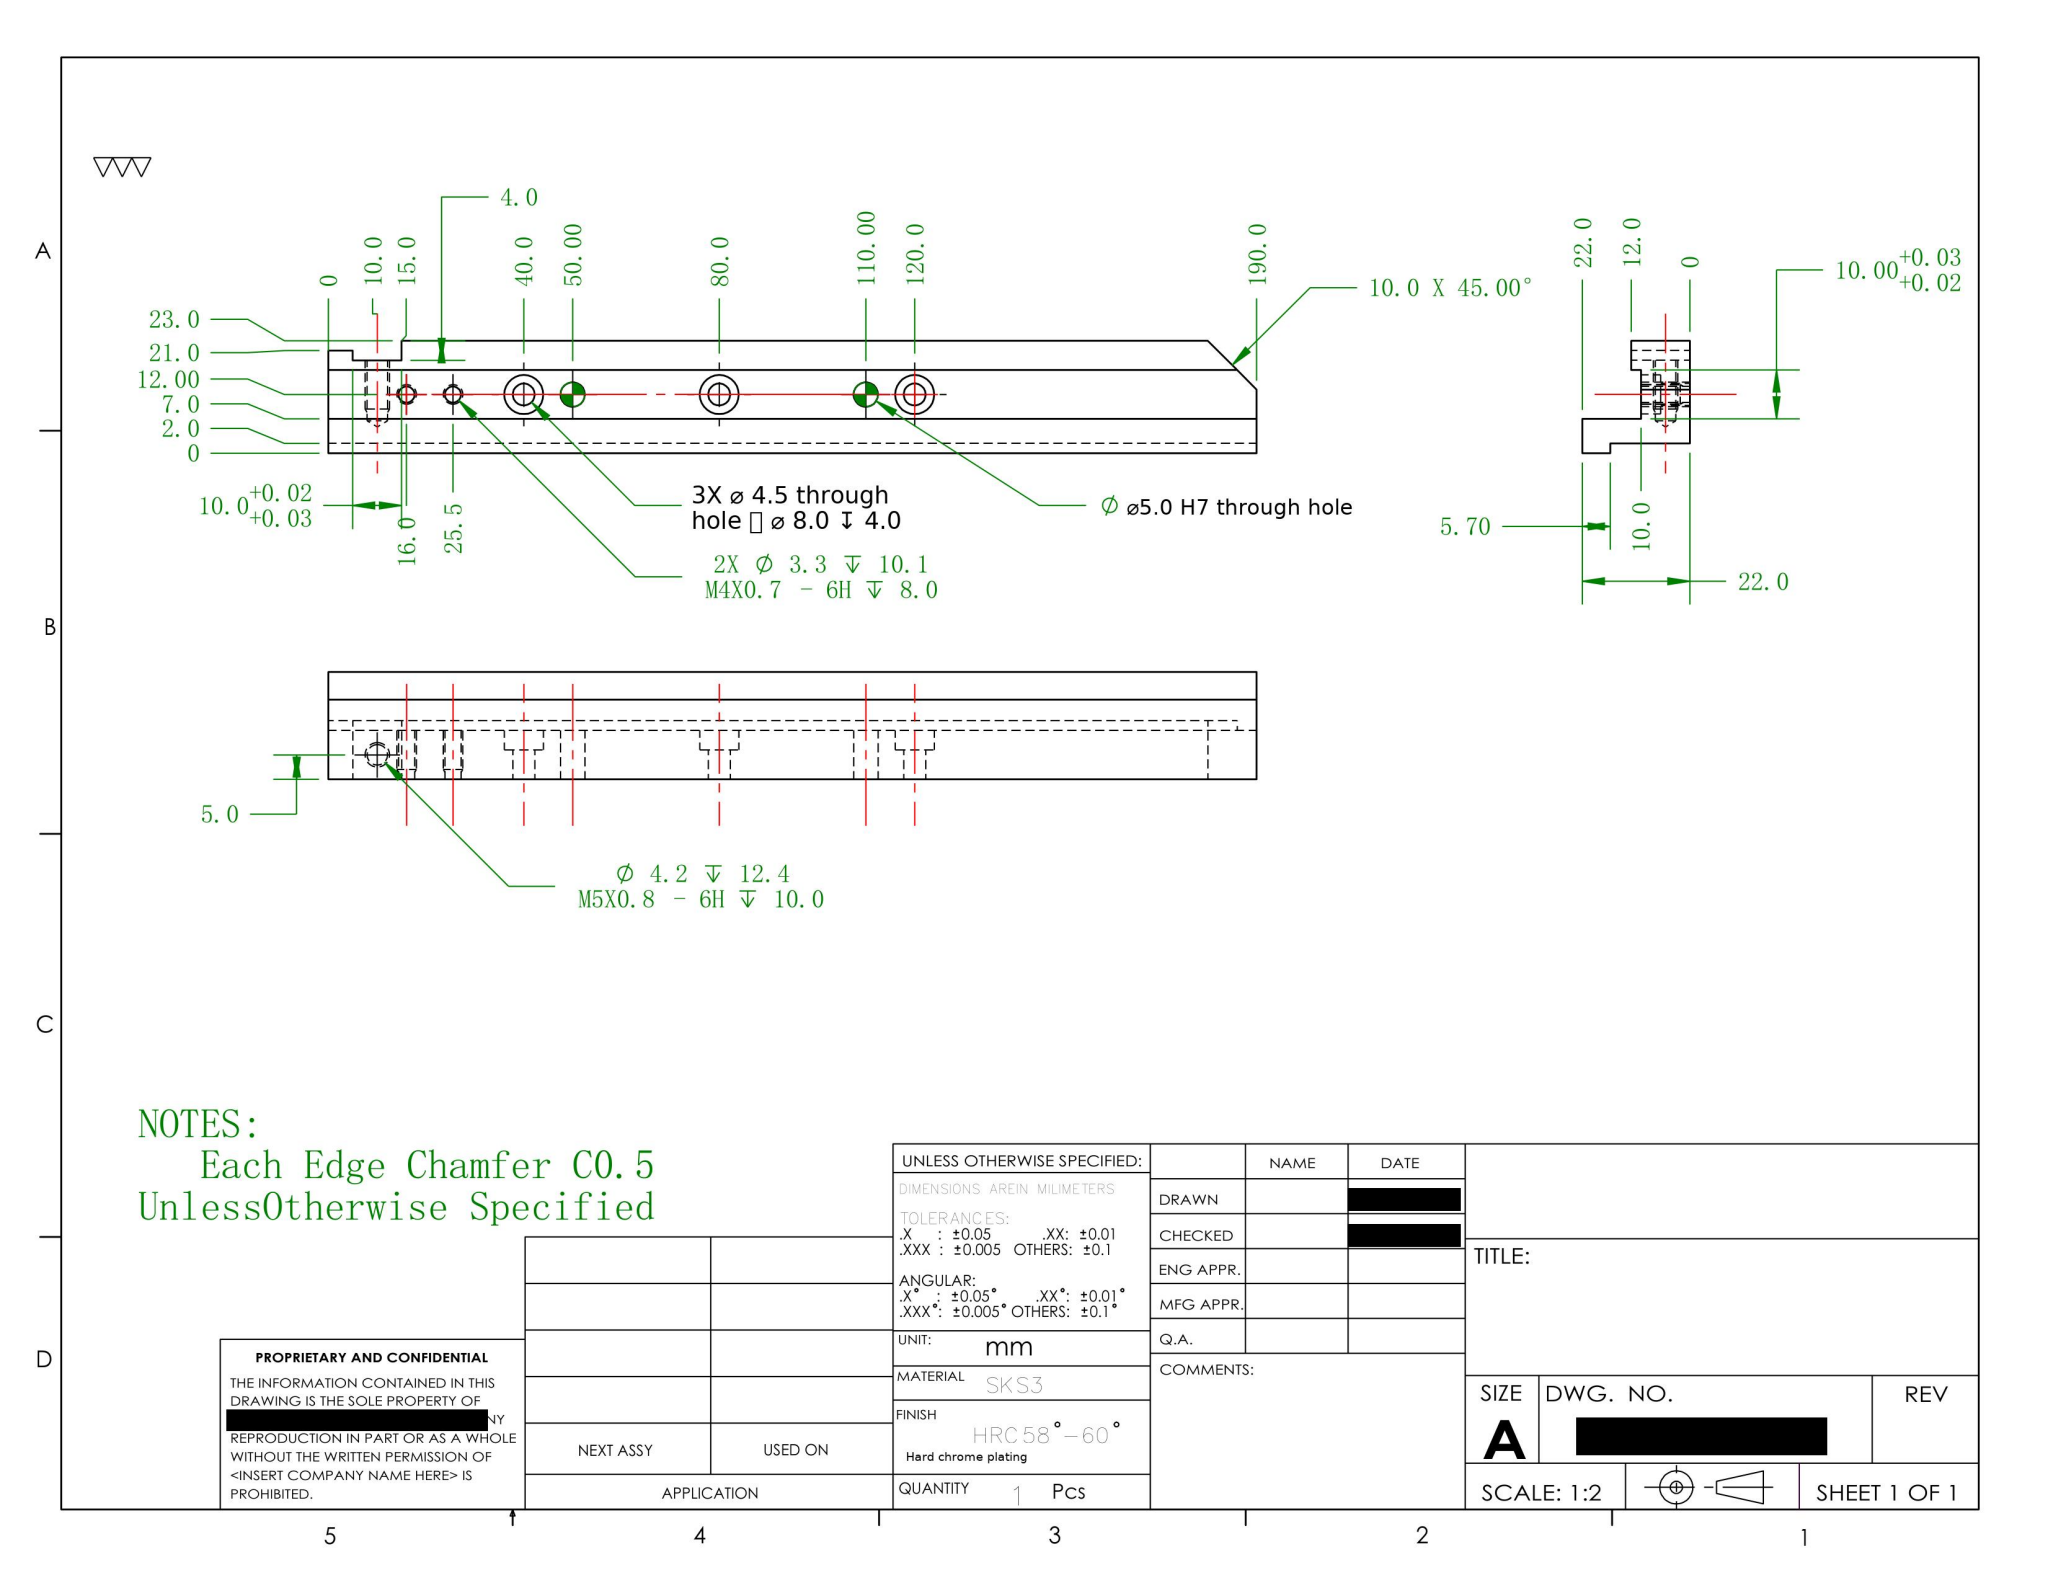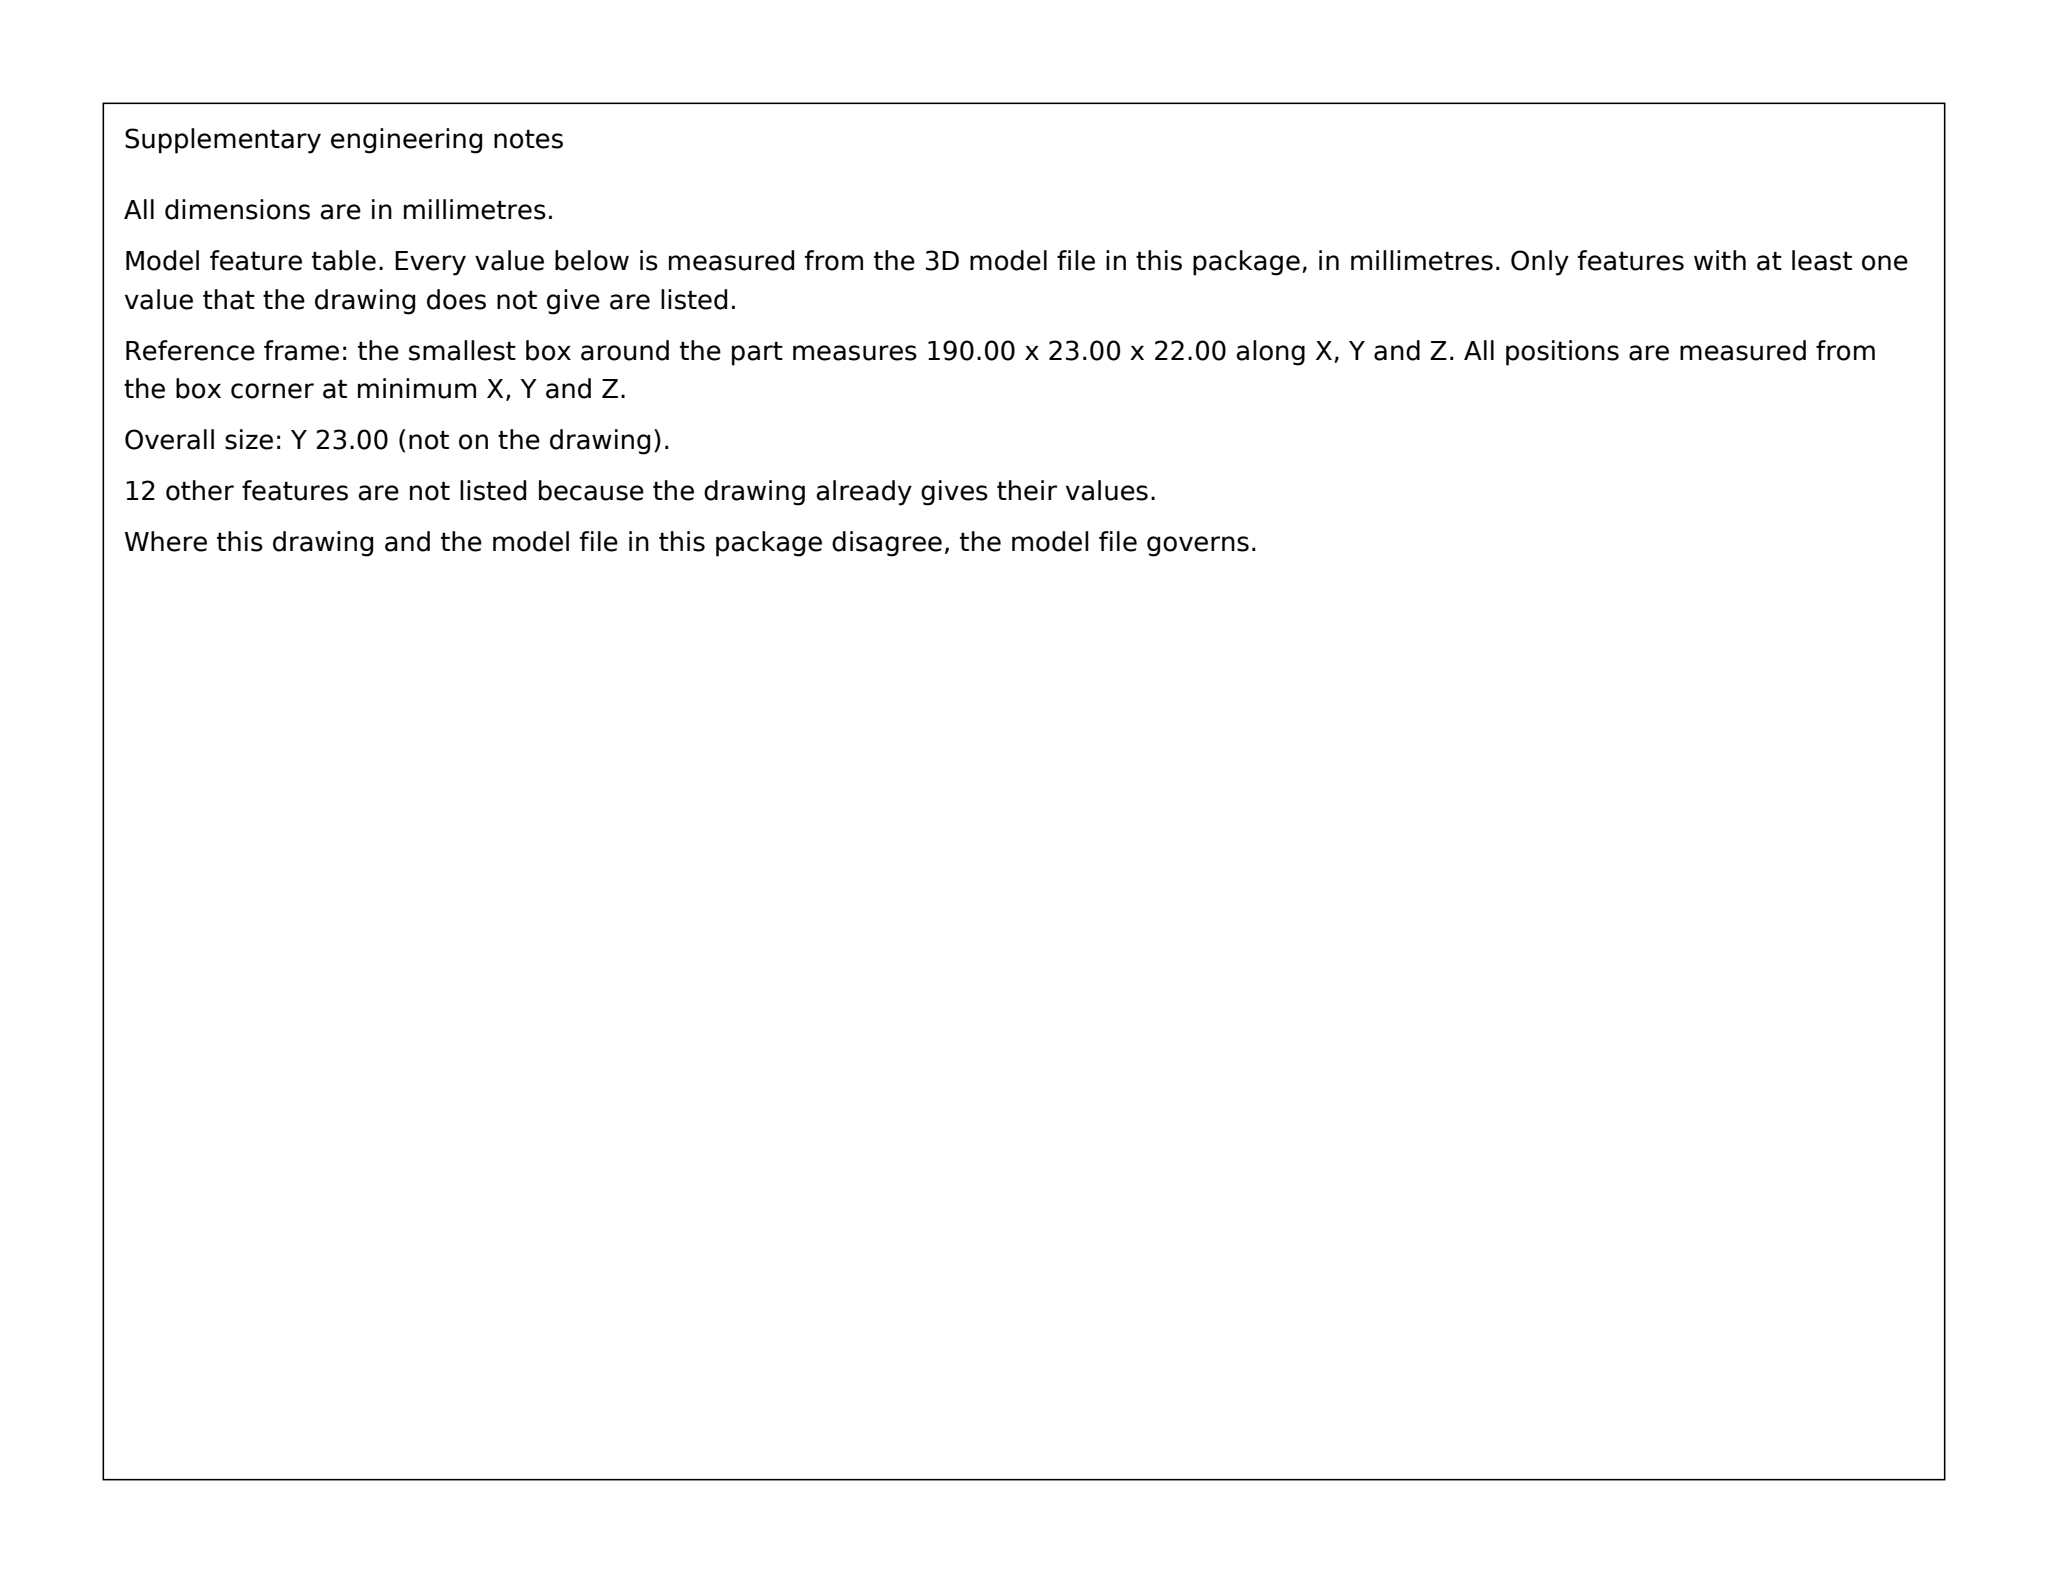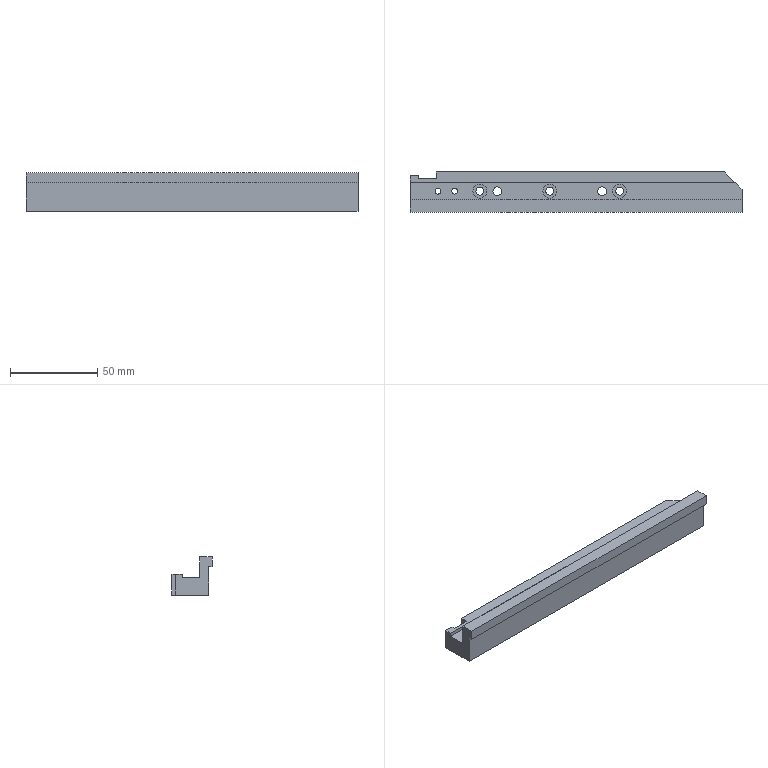Part | SolidWorks | mm | material SKS3 | 1 solid | 44 faces | box 190 x 23 x 22 mm | volume 52931 mm3 | cylinder 22 | plane 20 | cone 2 | commonest cylinder face diameters 8 x6 4.5 x6 5 x4 3.3 x4 4.2 x2
build123d program:
from build123d import *

# Parameters (mm, degrees)
SKETCH1_W                                            = 190
SKETCH1_H                                            = 16
EXTRUDE1_DEPTH                                       = 12
SKETCH5_W                                            = 190
SKETCH5_H                                            = 22
EXTRUDE2_DEPTH                                       = 5
SKETCH6_W                                            = 190
SKETCH6_H                                            = 4.9
EXTRUDE3_DEPTH                                       = 2
SKETCH7_W                                            = 190
SKETCH7_H                                            = 16
EXTRUDE4_DEPTH                                       = 2
SKETCH8_W                                            = 190
SKETCH8_H                                            = 6
EXTRUDE5_DEPTH                                       = 2
SKETCH9_W                                            = 15
SKETCH9_H                                            = 12
CUT_EXTRUDE2_DEPTH                                   = 2
SKETCH10_W                                           = 10
SKETCH10_H                                           = 12
EXTRUDE6_DEPTH                                       = 2
M5X0_8_TAPPED_HOLE1_D                                = 4.2
M5X0_8_TAPPED_HOLE1_DEPTH                            = 12.4
M5X0_8_TAPPED_HOLE1_TIP                              = 1.262
M4X0_7_TAPPED_HOLE3_D                                = 3.3
M4X0_7_TAPPED_HOLE3_DEPTH                            = 10.1
M4X0_7_TAPPED_HOLE3_TIP                              = 0.9914
CHAMFER2_SIZE                                        = 10
SKETCH17_R                                           = 2.5
CUT_EXTRUDE3_DEPTH                                   = 192.05
CYLINDRICAL_COUNTERSUNK_HOLE_FOR_M4_SOCK_D           = 4.5
CYLINDRICAL_COUNTERSUNK_HOLE_FOR_M4_SOCK_CBORE_D     = 8
CYLINDRICAL_COUNTERSUNK_HOLE_FOR_M4_SOCK_CBORE_DEPTH = 4
SKETCH20_W                                           = 190
SKETCH20_H                                           = 2
EXTRUDE7_DEPTH                                       = 3
SKETCH21_W                                           = 190
SKETCH21_H                                           = 2
CUT_EXTRUDE4_DEPTH                                   = 2.2


with BuildPart() as part:
    # Sketch1 → Extrude1 (new body)
    with BuildSketch(Plane.XY):
        with Locations((95, 8)):
            Rectangle(SKETCH1_W, SKETCH1_H)
    extrude(amount=EXTRUDE1_DEPTH)

    # Sketch5 → Extrude2 (add)
    with BuildSketch(Plane.XZ):
        with Locations((95, 11)):
            Rectangle(SKETCH5_W, SKETCH5_H)
    extrude(amount=EXTRUDE2_DEPTH)

    # Sketch6 → Extrude3 (add)
    with BuildSketch(Plane.XZ.offset(5)):
        with Locations((95, 19.55)):
            Rectangle(SKETCH6_W, SKETCH6_H)
    extrude(amount=EXTRUDE3_DEPTH)

    # Sketch7 → Extrude4 (cut)
    with BuildSketch(Plane.XY.offset(12)):
        with Locations((95, 8)):
            Rectangle(SKETCH7_W, SKETCH7_H)
    extrude(amount=-EXTRUDE4_DEPTH, mode=Mode.SUBTRACT)

    # Sketch8 → Extrude5 (add)
    with BuildSketch(Plane.XY.offset(10)):
        with Locations((95, 13)):
            Rectangle(SKETCH8_W, SKETCH8_H)
    extrude(amount=EXTRUDE5_DEPTH)

    # Sketch9 → Cut-Extrude2 (cut)
    with BuildSketch(Plane(origin=(0, 16, 0), x_dir=(1, 0, 0), z_dir=(0, 1, 0))):
        with Locations((7.5, -6)):
            Rectangle(SKETCH9_W, SKETCH9_H)
    extrude(amount=-CUT_EXTRUDE2_DEPTH, mode=Mode.SUBTRACT)

    # Sketch10 → Extrude6 (cut)
    with BuildSketch(Plane(origin=(0, 14, 0), x_dir=(1, 0, 0), z_dir=(0, 1, 0))):
        with Locations((10, -6)):
            Rectangle(SKETCH10_W, SKETCH10_H)
    extrude(amount=-EXTRUDE6_DEPTH, mode=Mode.SUBTRACT)

    # M5x0.8 Tapped Hole1
    with Locations(Plane(origin=(0, 12, 0), x_dir=(-1, 0, 0), z_dir=(0, 1, 0))):
        with Locations((-10, 5)):
            Hole(M5X0_8_TAPPED_HOLE1_D / 2, depth=M5X0_8_TAPPED_HOLE1_DEPTH)
            with Locations((0, 0, -(M5X0_8_TAPPED_HOLE1_DEPTH + M5X0_8_TAPPED_HOLE1_TIP / 2))):  # 118° drill point
                Cone(0, M5X0_8_TAPPED_HOLE1_D / 2, M5X0_8_TAPPED_HOLE1_TIP, mode=Mode.SUBTRACT)

    # M4x0.7 Tapped Hole3
    with Locations(Plane.XY.offset(10)):
        with Locations((16, 5), (25.5, 5)):
            Hole(M4X0_7_TAPPED_HOLE3_D / 2, depth=M4X0_7_TAPPED_HOLE3_DEPTH)
            with Locations((0, 0, -(M4X0_7_TAPPED_HOLE3_DEPTH + M4X0_7_TAPPED_HOLE3_TIP / 2))):  # 118° drill point
                Cone(0, M4X0_7_TAPPED_HOLE3_D / 2, M4X0_7_TAPPED_HOLE3_TIP, mode=Mode.SUBTRACT)

    # Chamfer2
    chamfer2_edges = [part.edges().sort_by_distance(p)[0] for p in [
        (190, 16, 6),
    ]]
    chamfer(chamfer2_edges, length=CHAMFER2_SIZE)

    # Sketch17 → Cut-Extrude3 (cut, through all)
    with BuildSketch(Plane.XY.offset(10)):
        with Locations((50, 5)):
            Circle(SKETCH17_R)
        with Locations((110, 5)):
            Circle(SKETCH17_R)
    extrude(amount=-CUT_EXTRUDE3_DEPTH, mode=Mode.SUBTRACT)

    # Cylindrical Countersunk Hole for M4 Sock (through all)
    with Locations(Plane.XY.offset(10)):
        with Locations((80, 5), (40, 5), (120, 5)):
            CounterBoreHole(CYLINDRICAL_COUNTERSUNK_HOLE_FOR_M4_SOCK_D / 2, CYLINDRICAL_COUNTERSUNK_HOLE_FOR_M4_SOCK_CBORE_D / 2, CYLINDRICAL_COUNTERSUNK_HOLE_FOR_M4_SOCK_CBORE_DEPTH)

    # Sketch20 → Extrude7 (add)
    with BuildSketch(Plane(origin=(0, 0, 17.1), x_dir=(-1, 0, 0), z_dir=(0, 0, -1))):
        with Locations((-95, -6)):
            Rectangle(SKETCH20_W, SKETCH20_H)
    extrude(amount=EXTRUDE7_DEPTH)

    # Sketch21 → Cut-Extrude4 (cut)
    with BuildSketch(Plane(origin=(0, 0, 14.1), x_dir=(-1, 0, 0), z_dir=(0, 0, -1))):
        with Locations((-95, -6)):
            Rectangle(SKETCH21_W, SKETCH21_H)
    extrude(amount=-CUT_EXTRUDE4_DEPTH, mode=Mode.SUBTRACT)


solid = part.part